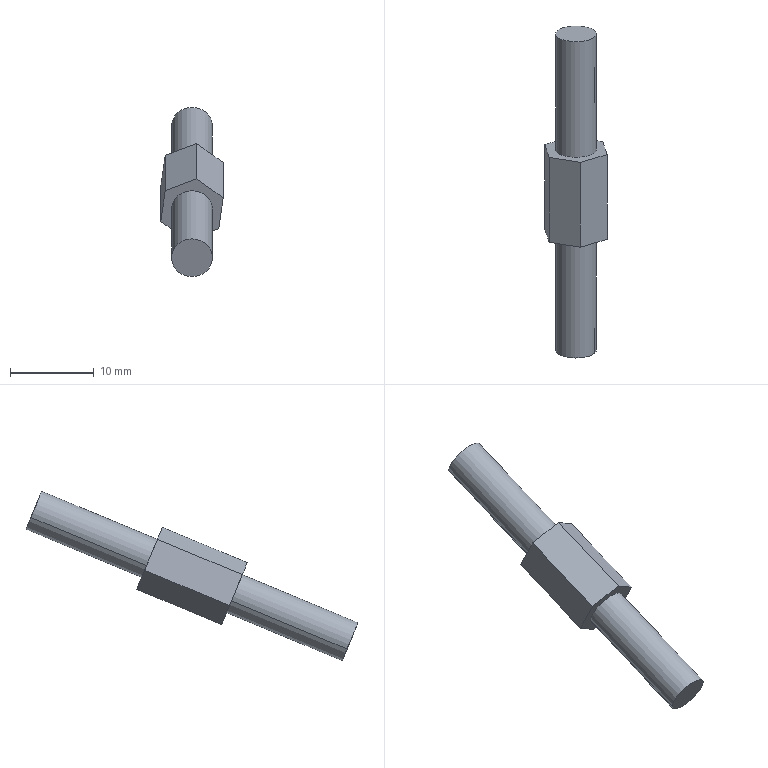Component | SolidWorks | 04-001Screw-1 | 1 solid | 14 faces | box 7.47 x 39.74 x 20.27 mm | volume 1033 mm3 | plane 10 | cylinder 4 | commonest cylinder face diameters 4.9 x4
STEP:
#1=CARTESIAN_POINT('',(0.2949,0.5363,3.574));
#2=VERTEX_POINT('',#1);
#3=CARTESIAN_POINT('',(0.1166,0.5645,3.506));
#4=VERTEX_POINT('',#3);
#5=CARTESIAN_POINT('',(0.2058,0.5504,3.54));
#6=DIRECTION('',(0.,0.9233,0.384));
#7=DIRECTION('',(0.9242,-0.1466,0.3526));
#8=AXIS2_PLACEMENT_3D('',#5,#6,#7);
#9=CIRCLE('',#8,0.09646);
#10=EDGE_CURVE('',#2,#4,#9,.T.);
#11=ORIENTED_EDGE('',*,*,#10,.T.);
#12=CARTESIAN_POINT('',(0.1166,1.11,3.733));
#13=VERTEX_POINT('',#12);
#14=CARTESIAN_POINT('',(0.1166,0.5645,3.506));
#15=DIRECTION('',(0.,0.9233,0.384));
#16=VECTOR('',#15,39.37);
#17=LINE('',#14,#16);
#18=EDGE_CURVE('',#4,#13,#17,.T.);
#19=ORIENTED_EDGE('',*,*,#18,.T.);
#20=CARTESIAN_POINT('',(0.2949,1.082,3.801));
#21=VERTEX_POINT('',#20);
#22=CARTESIAN_POINT('',(0.2058,1.096,3.767));
#23=DIRECTION('',(0.,0.9233,0.384));
#24=DIRECTION('',(0.9242,-0.1466,0.3526));
#25=AXIS2_PLACEMENT_3D('',#22,#23,#24);
#26=CIRCLE('',#25,0.09646);
#27=EDGE_CURVE('',#21,#13,#26,.T.);
#28=ORIENTED_EDGE('',*,*,#27,.F.);
#29=CARTESIAN_POINT('',(0.2949,0.5363,3.574));
#30=DIRECTION('',(0.,0.9233,0.384));
#31=VECTOR('',#30,39.37);
#32=LINE('',#29,#31);
#33=EDGE_CURVE('',#2,#21,#32,.T.);
#34=ORIENTED_EDGE('',*,*,#33,.F.);
#35=EDGE_LOOP('',(#11,#19,#28,#34));
#36=FACE_OUTER_BOUND('',#35,.T.);
#37=CARTESIAN_POINT('',(0.2058,0.5504,3.54));
#38=DIRECTION('',(0.,0.9233,0.384));
#39=DIRECTION('',(0.9242,-0.1466,0.3526));
#40=AXIS2_PLACEMENT_3D('',#37,#38,#39);
#41=CYLINDRICAL_SURFACE('',#40,0.09646);
#42=ADVANCED_FACE('',(#36),#41,.T.);
#43=CARTESIAN_POINT('',(0.2949,2.027,4.194));
#44=VERTEX_POINT('',#43);
#45=CARTESIAN_POINT('',(0.1166,2.055,4.126));
#46=VERTEX_POINT('',#45);
#47=CARTESIAN_POINT('',(0.2058,2.041,4.16));
#48=DIRECTION('',(0.,0.9233,0.384));
#49=DIRECTION('',(0.9242,-0.1466,0.3526));
#50=AXIS2_PLACEMENT_3D('',#47,#48,#49);
#51=CIRCLE('',#50,0.09646);
#52=EDGE_CURVE('',#44,#46,#51,.T.);
#53=ORIENTED_EDGE('',*,*,#52,.F.);
#54=CARTESIAN_POINT('',(0.2949,1.481,3.968));
#55=VERTEX_POINT('',#54);
#56=CARTESIAN_POINT('',(0.2949,2.027,4.194));
#57=DIRECTION('',(-0.,-0.9233,-0.384));
#58=VECTOR('',#57,39.37);
#59=LINE('',#56,#58);
#60=EDGE_CURVE('',#44,#55,#59,.T.);
#61=ORIENTED_EDGE('',*,*,#60,.T.);
#62=CARTESIAN_POINT('',(0.1166,1.51,3.9));
#63=VERTEX_POINT('',#62);
#64=CARTESIAN_POINT('',(0.2058,1.496,3.934));
#65=DIRECTION('',(0.,0.9233,0.384));
#66=DIRECTION('',(0.9242,-0.1466,0.3526));
#67=AXIS2_PLACEMENT_3D('',#64,#65,#66);
#68=CIRCLE('',#67,0.09646);
#69=EDGE_CURVE('',#55,#63,#68,.T.);
#70=ORIENTED_EDGE('',*,*,#69,.T.);
#71=CARTESIAN_POINT('',(0.1166,2.055,4.126));
#72=DIRECTION('',(-0.,-0.9233,-0.384));
#73=VECTOR('',#72,39.37);
#74=LINE('',#71,#73);
#75=EDGE_CURVE('',#46,#63,#74,.T.);
#76=ORIENTED_EDGE('',*,*,#75,.F.);
#77=EDGE_LOOP('',(#53,#61,#70,#76));
#78=FACE_OUTER_BOUND('',#77,.T.);
#79=CARTESIAN_POINT('',(0.2058,2.041,4.16));
#80=DIRECTION('',(-0.,-0.9233,-0.384));
#81=DIRECTION('',(-0.9242,0.1466,-0.3526));
#82=AXIS2_PLACEMENT_3D('',#79,#80,#81);
#83=CYLINDRICAL_SURFACE('',#82,0.09646);
#84=ADVANCED_FACE('',(#78),#83,.T.);
#85=CARTESIAN_POINT('',(0.07962,1.458,4.023));
#86=VERTEX_POINT('',#85);
#87=CARTESIAN_POINT('',(0.2267,1.435,4.079));
#88=VERTEX_POINT('',#87);
#89=CARTESIAN_POINT('',(0.07962,1.458,4.023));
#90=DIRECTION('',(0.9242,-0.1466,0.3526));
#91=VECTOR('',#90,39.37);
#92=LINE('',#89,#91);
#93=EDGE_CURVE('',#86,#88,#92,.T.);
#94=ORIENTED_EDGE('',*,*,#93,.T.);
#95=CARTESIAN_POINT('',(0.3528,1.472,3.99));
#96=VERTEX_POINT('',#95);
#97=CARTESIAN_POINT('',(0.2267,1.435,4.079));
#98=DIRECTION('',(0.7928,0.2341,-0.5627));
#99=VECTOR('',#98,39.37);
#100=LINE('',#97,#99);
#101=EDGE_CURVE('',#88,#96,#100,.T.);
#102=ORIENTED_EDGE('',*,*,#101,.T.);
#103=CARTESIAN_POINT('',(0.3319,1.533,3.844));
#104=VERTEX_POINT('',#103);
#105=CARTESIAN_POINT('',(0.3528,1.472,3.99));
#106=DIRECTION('',(-0.1314,0.3807,-0.9153));
#107=VECTOR('',#106,39.37);
#108=LINE('',#105,#107);
#109=EDGE_CURVE('',#96,#104,#108,.T.);
#110=ORIENTED_EDGE('',*,*,#109,.T.);
#111=CARTESIAN_POINT('',(0.1849,1.556,3.788));
#112=VERTEX_POINT('',#111);
#113=CARTESIAN_POINT('',(0.3319,1.533,3.844));
#114=DIRECTION('',(-0.9242,0.1466,-0.3526));
#115=VECTOR('',#114,39.37);
#116=LINE('',#113,#115);
#117=EDGE_CURVE('',#104,#112,#116,.T.);
#118=ORIENTED_EDGE('',*,*,#117,.T.);
#119=CARTESIAN_POINT('',(0.05871,1.519,3.877));
#120=VERTEX_POINT('',#119);
#121=CARTESIAN_POINT('',(0.1849,1.556,3.788));
#122=DIRECTION('',(-0.7928,-0.2341,0.5627));
#123=VECTOR('',#122,39.37);
#124=LINE('',#121,#123);
#125=EDGE_CURVE('',#112,#120,#124,.T.);
#126=ORIENTED_EDGE('',*,*,#125,.T.);
#127=CARTESIAN_POINT('',(0.05871,1.519,3.877));
#128=DIRECTION('',(0.1314,-0.3807,0.9153));
#129=VECTOR('',#128,39.37);
#130=LINE('',#127,#129);
#131=EDGE_CURVE('',#120,#86,#130,.T.);
#132=ORIENTED_EDGE('',*,*,#131,.T.);
#133=EDGE_LOOP('',(#94,#102,#110,#118,#126,#132));
#134=FACE_OUTER_BOUND('',#133,.T.);
#135=CARTESIAN_POINT('',(0.2058,1.496,3.934));
#136=DIRECTION('',(0.,0.9233,0.384));
#137=DIRECTION('',(0.9242,-0.1466,0.3526));
#138=AXIS2_PLACEMENT_3D('',#135,#136,#137);
#139=CIRCLE('',#138,0.09646);
#140=EDGE_CURVE('',#63,#55,#139,.T.);
#141=ORIENTED_EDGE('',*,*,#140,.F.);
#142=ORIENTED_EDGE('',*,*,#69,.F.);
#143=EDGE_LOOP('',(#141,#142));
#144=FACE_BOUND('',#143,.T.);
#145=CARTESIAN_POINT('',(0.2058,1.496,3.934));
#146=DIRECTION('',(0.,0.9233,0.384));
#147=DIRECTION('',(0.9242,-0.1466,0.3526));
#148=AXIS2_PLACEMENT_3D('',#145,#146,#147);
#149=PLANE('',#148);
#150=ADVANCED_FACE('',(#134,#144),#149,.T.);
#151=CARTESIAN_POINT('',(0.07962,1.058,3.857));
#152=VERTEX_POINT('',#151);
#153=CARTESIAN_POINT('',(0.2267,1.035,3.913));
#154=VERTEX_POINT('',#153);
#155=CARTESIAN_POINT('',(0.07962,1.058,3.857));
#156=DIRECTION('',(0.9242,-0.1466,0.3526));
#157=VECTOR('',#156,39.37);
#158=LINE('',#155,#157);
#159=EDGE_CURVE('',#152,#154,#158,.T.);
#160=ORIENTED_EDGE('',*,*,#159,.T.);
#161=CARTESIAN_POINT('',(0.2267,1.435,4.079));
#162=DIRECTION('',(-0.,-0.9233,-0.384));
#163=VECTOR('',#162,39.37);
#164=LINE('',#161,#163);
#165=EDGE_CURVE('',#88,#154,#164,.T.);
#166=ORIENTED_EDGE('',*,*,#165,.F.);
#167=ORIENTED_EDGE('',*,*,#93,.F.);
#168=CARTESIAN_POINT('',(0.07962,1.458,4.023));
#169=DIRECTION('',(-0.,-0.9233,-0.384));
#170=VECTOR('',#169,39.37);
#171=LINE('',#168,#170);
#172=EDGE_CURVE('',#86,#152,#171,.T.);
#173=ORIENTED_EDGE('',*,*,#172,.T.);
#174=EDGE_LOOP('',(#160,#166,#167,#173));
#175=FACE_OUTER_BOUND('',#174,.T.);
#176=CARTESIAN_POINT('',(0.07962,1.458,4.023));
#177=DIRECTION('',(0.3818,0.3549,-0.8534));
#178=DIRECTION('',(-0.9242,0.1466,-0.3526));
#179=AXIS2_PLACEMENT_3D('',#176,#177,#178);
#180=PLANE('',#179);
#181=ADVANCED_FACE('',(#175),#180,.F.);
#182=CARTESIAN_POINT('',(0.3528,1.072,3.823));
#183=VERTEX_POINT('',#182);
#184=CARTESIAN_POINT('',(0.2267,1.035,3.913));
#185=DIRECTION('',(0.7928,0.2341,-0.5627));
#186=VECTOR('',#185,39.37);
#187=LINE('',#184,#186);
#188=EDGE_CURVE('',#154,#183,#187,.T.);
#189=ORIENTED_EDGE('',*,*,#188,.T.);
#190=CARTESIAN_POINT('',(0.3528,1.472,3.99));
#191=DIRECTION('',(-0.,-0.9233,-0.384));
#192=VECTOR('',#191,39.37);
#193=LINE('',#190,#192);
#194=EDGE_CURVE('',#96,#183,#193,.T.);
#195=ORIENTED_EDGE('',*,*,#194,.F.);
#196=ORIENTED_EDGE('',*,*,#101,.F.);
#197=ORIENTED_EDGE('',*,*,#165,.T.);
#198=EDGE_LOOP('',(#189,#195,#196,#197));
#199=FACE_OUTER_BOUND('',#198,.T.);
#200=CARTESIAN_POINT('',(0.2267,1.435,4.079));
#201=DIRECTION('',(-0.6095,0.3045,-0.732));
#202=DIRECTION('',(-0.7928,-0.2341,0.5627));
#203=AXIS2_PLACEMENT_3D('',#200,#201,#202);
#204=PLANE('',#203);
#205=ADVANCED_FACE('',(#199),#204,.F.);
#206=CARTESIAN_POINT('',(0.3319,1.133,3.678));
#207=VERTEX_POINT('',#206);
#208=CARTESIAN_POINT('',(0.3528,1.072,3.823));
#209=DIRECTION('',(-0.1314,0.3807,-0.9153));
#210=VECTOR('',#209,39.37);
#211=LINE('',#208,#210);
#212=EDGE_CURVE('',#183,#207,#211,.T.);
#213=ORIENTED_EDGE('',*,*,#212,.T.);
#214=CARTESIAN_POINT('',(0.3319,1.533,3.844));
#215=DIRECTION('',(-0.,-0.9233,-0.384));
#216=VECTOR('',#215,39.37);
#217=LINE('',#214,#216);
#218=EDGE_CURVE('',#104,#207,#217,.T.);
#219=ORIENTED_EDGE('',*,*,#218,.F.);
#220=ORIENTED_EDGE('',*,*,#109,.F.);
#221=ORIENTED_EDGE('',*,*,#194,.T.);
#222=EDGE_LOOP('',(#213,#219,#220,#221));
#223=FACE_OUTER_BOUND('',#222,.T.);
#224=CARTESIAN_POINT('',(0.3528,1.472,3.99));
#225=DIRECTION('',(-0.9913,-0.05047,0.1213));
#226=DIRECTION('',(0.1314,-0.3807,0.9153));
#227=AXIS2_PLACEMENT_3D('',#224,#225,#226);
#228=PLANE('',#227);
#229=ADVANCED_FACE('',(#223),#228,.F.);
#230=CARTESIAN_POINT('',(0.1849,1.156,3.622));
#231=VERTEX_POINT('',#230);
#232=CARTESIAN_POINT('',(0.3319,1.133,3.678));
#233=DIRECTION('',(-0.9242,0.1466,-0.3526));
#234=VECTOR('',#233,39.37);
#235=LINE('',#232,#234);
#236=EDGE_CURVE('',#207,#231,#235,.T.);
#237=ORIENTED_EDGE('',*,*,#236,.T.);
#238=CARTESIAN_POINT('',(0.1849,1.556,3.788));
#239=DIRECTION('',(-0.,-0.9233,-0.384));
#240=VECTOR('',#239,39.37);
#241=LINE('',#238,#240);
#242=EDGE_CURVE('',#112,#231,#241,.T.);
#243=ORIENTED_EDGE('',*,*,#242,.F.);
#244=ORIENTED_EDGE('',*,*,#117,.F.);
#245=ORIENTED_EDGE('',*,*,#218,.T.);
#246=EDGE_LOOP('',(#237,#243,#244,#245));
#247=FACE_OUTER_BOUND('',#246,.T.);
#248=CARTESIAN_POINT('',(0.3319,1.533,3.844));
#249=DIRECTION('',(-0.3818,-0.3549,0.8534));
#250=DIRECTION('',(0.9242,-0.1466,0.3526));
#251=AXIS2_PLACEMENT_3D('',#248,#249,#250);
#252=PLANE('',#251);
#253=ADVANCED_FACE('',(#247),#252,.F.);
#254=CARTESIAN_POINT('',(0.05871,1.119,3.711));
#255=VERTEX_POINT('',#254);
#256=CARTESIAN_POINT('',(0.1849,1.156,3.622));
#257=DIRECTION('',(-0.7928,-0.2341,0.5627));
#258=VECTOR('',#257,39.37);
#259=LINE('',#256,#258);
#260=EDGE_CURVE('',#231,#255,#259,.T.);
#261=ORIENTED_EDGE('',*,*,#260,.T.);
#262=CARTESIAN_POINT('',(0.05871,1.519,3.877));
#263=DIRECTION('',(-0.,-0.9233,-0.384));
#264=VECTOR('',#263,39.37);
#265=LINE('',#262,#264);
#266=EDGE_CURVE('',#120,#255,#265,.T.);
#267=ORIENTED_EDGE('',*,*,#266,.F.);
#268=ORIENTED_EDGE('',*,*,#125,.F.);
#269=ORIENTED_EDGE('',*,*,#242,.T.);
#270=EDGE_LOOP('',(#261,#267,#268,#269));
#271=FACE_OUTER_BOUND('',#270,.T.);
#272=CARTESIAN_POINT('',(0.1849,1.556,3.788));
#273=DIRECTION('',(0.6095,-0.3045,0.732));
#274=DIRECTION('',(0.7928,0.2341,-0.5627));
#275=AXIS2_PLACEMENT_3D('',#272,#273,#274);
#276=PLANE('',#275);
#277=ADVANCED_FACE('',(#271),#276,.F.);
#278=CARTESIAN_POINT('',(0.05871,1.119,3.711));
#279=DIRECTION('',(0.1314,-0.3807,0.9153));
#280=VECTOR('',#279,39.37);
#281=LINE('',#278,#280);
#282=EDGE_CURVE('',#255,#152,#281,.T.);
#283=ORIENTED_EDGE('',*,*,#282,.T.);
#284=ORIENTED_EDGE('',*,*,#172,.F.);
#285=ORIENTED_EDGE('',*,*,#131,.F.);
#286=ORIENTED_EDGE('',*,*,#266,.T.);
#287=EDGE_LOOP('',(#283,#284,#285,#286));
#288=FACE_OUTER_BOUND('',#287,.T.);
#289=CARTESIAN_POINT('',(0.05871,1.519,3.877));
#290=DIRECTION('',(0.9913,0.05047,-0.1213));
#291=DIRECTION('',(-0.1314,0.3807,-0.9153));
#292=AXIS2_PLACEMENT_3D('',#289,#290,#291);
#293=PLANE('',#292);
#294=ADVANCED_FACE('',(#288),#293,.F.);
#295=ORIENTED_EDGE('',*,*,#27,.T.);
#296=CARTESIAN_POINT('',(0.2058,1.096,3.767));
#297=DIRECTION('',(0.,0.9233,0.384));
#298=DIRECTION('',(0.9242,-0.1466,0.3526));
#299=AXIS2_PLACEMENT_3D('',#296,#297,#298);
#300=CIRCLE('',#299,0.09646);
#301=EDGE_CURVE('',#13,#21,#300,.T.);
#302=ORIENTED_EDGE('',*,*,#301,.T.);
#303=EDGE_LOOP('',(#295,#302));
#304=FACE_BOUND('',#303,.T.);
#305=ORIENTED_EDGE('',*,*,#159,.F.);
#306=ORIENTED_EDGE('',*,*,#282,.F.);
#307=ORIENTED_EDGE('',*,*,#260,.F.);
#308=ORIENTED_EDGE('',*,*,#236,.F.);
#309=ORIENTED_EDGE('',*,*,#212,.F.);
#310=ORIENTED_EDGE('',*,*,#188,.F.);
#311=EDGE_LOOP('',(#305,#306,#307,#308,#309,#310));
#312=FACE_OUTER_BOUND('',#311,.T.);
#313=CARTESIAN_POINT('',(0.2058,1.096,3.767));
#314=DIRECTION('',(0.,0.9233,0.384));
#315=DIRECTION('',(0.9242,-0.1466,0.3526));
#316=AXIS2_PLACEMENT_3D('',#313,#314,#315);
#317=PLANE('',#316);
#318=ADVANCED_FACE('',(#304,#312),#317,.F.);
#319=ORIENTED_EDGE('',*,*,#60,.F.);
#320=CARTESIAN_POINT('',(0.2058,2.041,4.16));
#321=DIRECTION('',(0.,0.9233,0.384));
#322=DIRECTION('',(0.9242,-0.1466,0.3526));
#323=AXIS2_PLACEMENT_3D('',#320,#321,#322);
#324=CIRCLE('',#323,0.09646);
#325=EDGE_CURVE('',#46,#44,#324,.T.);
#326=ORIENTED_EDGE('',*,*,#325,.F.);
#327=ORIENTED_EDGE('',*,*,#75,.T.);
#328=ORIENTED_EDGE('',*,*,#140,.T.);
#329=EDGE_LOOP('',(#319,#326,#327,#328));
#330=FACE_OUTER_BOUND('',#329,.T.);
#331=CARTESIAN_POINT('',(0.2058,2.041,4.16));
#332=DIRECTION('',(-0.,-0.9233,-0.384));
#333=DIRECTION('',(-0.9242,0.1466,-0.3526));
#334=AXIS2_PLACEMENT_3D('',#331,#332,#333);
#335=CYLINDRICAL_SURFACE('',#334,0.09646);
#336=ADVANCED_FACE('',(#330),#335,.T.);
#337=ORIENTED_EDGE('',*,*,#325,.T.);
#338=ORIENTED_EDGE('',*,*,#52,.T.);
#339=EDGE_LOOP('',(#337,#338));
#340=FACE_OUTER_BOUND('',#339,.T.);
#341=CARTESIAN_POINT('',(0.2058,2.041,4.16));
#342=DIRECTION('',(0.,0.9233,0.384));
#343=DIRECTION('',(0.9242,-0.1466,0.3526));
#344=AXIS2_PLACEMENT_3D('',#341,#342,#343);
#345=PLANE('',#344);
#346=ADVANCED_FACE('',(#340),#345,.T.);
#347=ORIENTED_EDGE('',*,*,#18,.F.);
#348=CARTESIAN_POINT('',(0.2058,0.5504,3.54));
#349=DIRECTION('',(0.,0.9233,0.384));
#350=DIRECTION('',(0.9242,-0.1466,0.3526));
#351=AXIS2_PLACEMENT_3D('',#348,#349,#350);
#352=CIRCLE('',#351,0.09646);
#353=EDGE_CURVE('',#4,#2,#352,.T.);
#354=ORIENTED_EDGE('',*,*,#353,.T.);
#355=ORIENTED_EDGE('',*,*,#33,.T.);
#356=ORIENTED_EDGE('',*,*,#301,.F.);
#357=EDGE_LOOP('',(#347,#354,#355,#356));
#358=FACE_OUTER_BOUND('',#357,.T.);
#359=CARTESIAN_POINT('',(0.2058,0.5504,3.54));
#360=DIRECTION('',(0.,0.9233,0.384));
#361=DIRECTION('',(0.9242,-0.1466,0.3526));
#362=AXIS2_PLACEMENT_3D('',#359,#360,#361);
#363=CYLINDRICAL_SURFACE('',#362,0.09646);
#364=ADVANCED_FACE('',(#358),#363,.T.);
#365=ORIENTED_EDGE('',*,*,#10,.F.);
#366=ORIENTED_EDGE('',*,*,#353,.F.);
#367=EDGE_LOOP('',(#365,#366));
#368=FACE_OUTER_BOUND('',#367,.T.);
#369=CARTESIAN_POINT('',(0.2058,0.5504,3.54));
#370=DIRECTION('',(-0.,-0.9233,-0.384));
#371=DIRECTION('',(0.9242,-0.1466,0.3526));
#372=AXIS2_PLACEMENT_3D('',#369,#370,#371);
#373=PLANE('',#372);
#374=ADVANCED_FACE('',(#368),#373,.T.);
#375=CLOSED_SHELL('',(#42,#84,#150,#181,#205,#229,#253,#277,#294,#318,#336,#346,#364,#374));
#376=MANIFOLD_SOLID_BREP('',#375);
#377=CARTESIAN_POINT('',(0.,0.,0.));
#378=DIRECTION('',(0.,0.,1.));
#379=DIRECTION('',(1.,0.,0.));
#380=AXIS2_PLACEMENT_3D('',#377,#378,#379);
#381=(LENGTH_UNIT()NAMED_UNIT(*)SI_UNIT($,.METRE.));
#382=LENGTH_MEASURE_WITH_UNIT(LENGTH_MEASURE(0.0254),#381);
#383=DIMENSIONAL_EXPONENTS(1.,0.,0.,0.,0.,0.,0.);
#384=(CONVERSION_BASED_UNIT('',#382)LENGTH_UNIT()NAMED_UNIT(#383));
#385=UNCERTAINTY_MEASURE_WITH_UNIT(LENGTH_MEASURE(0.00001),#384,'','');
#386=(NAMED_UNIT(*)PLANE_ANGLE_UNIT()SI_UNIT($,.RADIAN.));
#387=(NAMED_UNIT(*)SI_UNIT($,.STERADIAN.)SOLID_ANGLE_UNIT());
#388=(GEOMETRIC_REPRESENTATION_CONTEXT(3)GLOBAL_UNCERTAINTY_ASSIGNED_CONTEXT((#385))GLOBAL_UNIT_ASSIGNED_CONTEXT((#384,#386,#387))REPRESENTATION_CONTEXT('',''));
#389=ADVANCED_BREP_SHAPE_REPRESENTATION('',(#376,#380),#388);
#390=COLOUR_RGB('',0.7922,0.8196,0.9333);
#391=FILL_AREA_STYLE_COLOUR('',#390);
#392=FILL_AREA_STYLE('',(#391));
#393=SURFACE_STYLE_FILL_AREA(#392);
#394=SURFACE_SIDE_STYLE('',(#393));
#395=SURFACE_STYLE_USAGE(.BOTH.,#394);
#396=PRESENTATION_STYLE_ASSIGNMENT((#395));
#397=STYLED_ITEM('',(#396),#376);
#398=PRESENTATION_LAYER_ASSIGNMENT('','',(#397));
#399=(LENGTH_UNIT()NAMED_UNIT(*)SI_UNIT($,.METRE.));
#400=LENGTH_MEASURE_WITH_UNIT(LENGTH_MEASURE(0.0254),#399);
#401=DIMENSIONAL_EXPONENTS(1.,0.,0.,0.,0.,0.,0.);
#402=(CONVERSION_BASED_UNIT('',#400)LENGTH_UNIT()NAMED_UNIT(#401));
#403=UNCERTAINTY_MEASURE_WITH_UNIT(LENGTH_MEASURE(0.00001),#402,'','');
#404=(NAMED_UNIT(*)PLANE_ANGLE_UNIT()SI_UNIT($,.RADIAN.));
#405=(NAMED_UNIT(*)SI_UNIT($,.STERADIAN.)SOLID_ANGLE_UNIT());
#406=(GEOMETRIC_REPRESENTATION_CONTEXT(3)GLOBAL_UNCERTAINTY_ASSIGNED_CONTEXT((#403))GLOBAL_UNIT_ASSIGNED_CONTEXT((#402,#404,#405))REPRESENTATION_CONTEXT('',''));
#407=MECHANICAL_DESIGN_GEOMETRIC_PRESENTATION_REPRESENTATION('',(#397),#406);